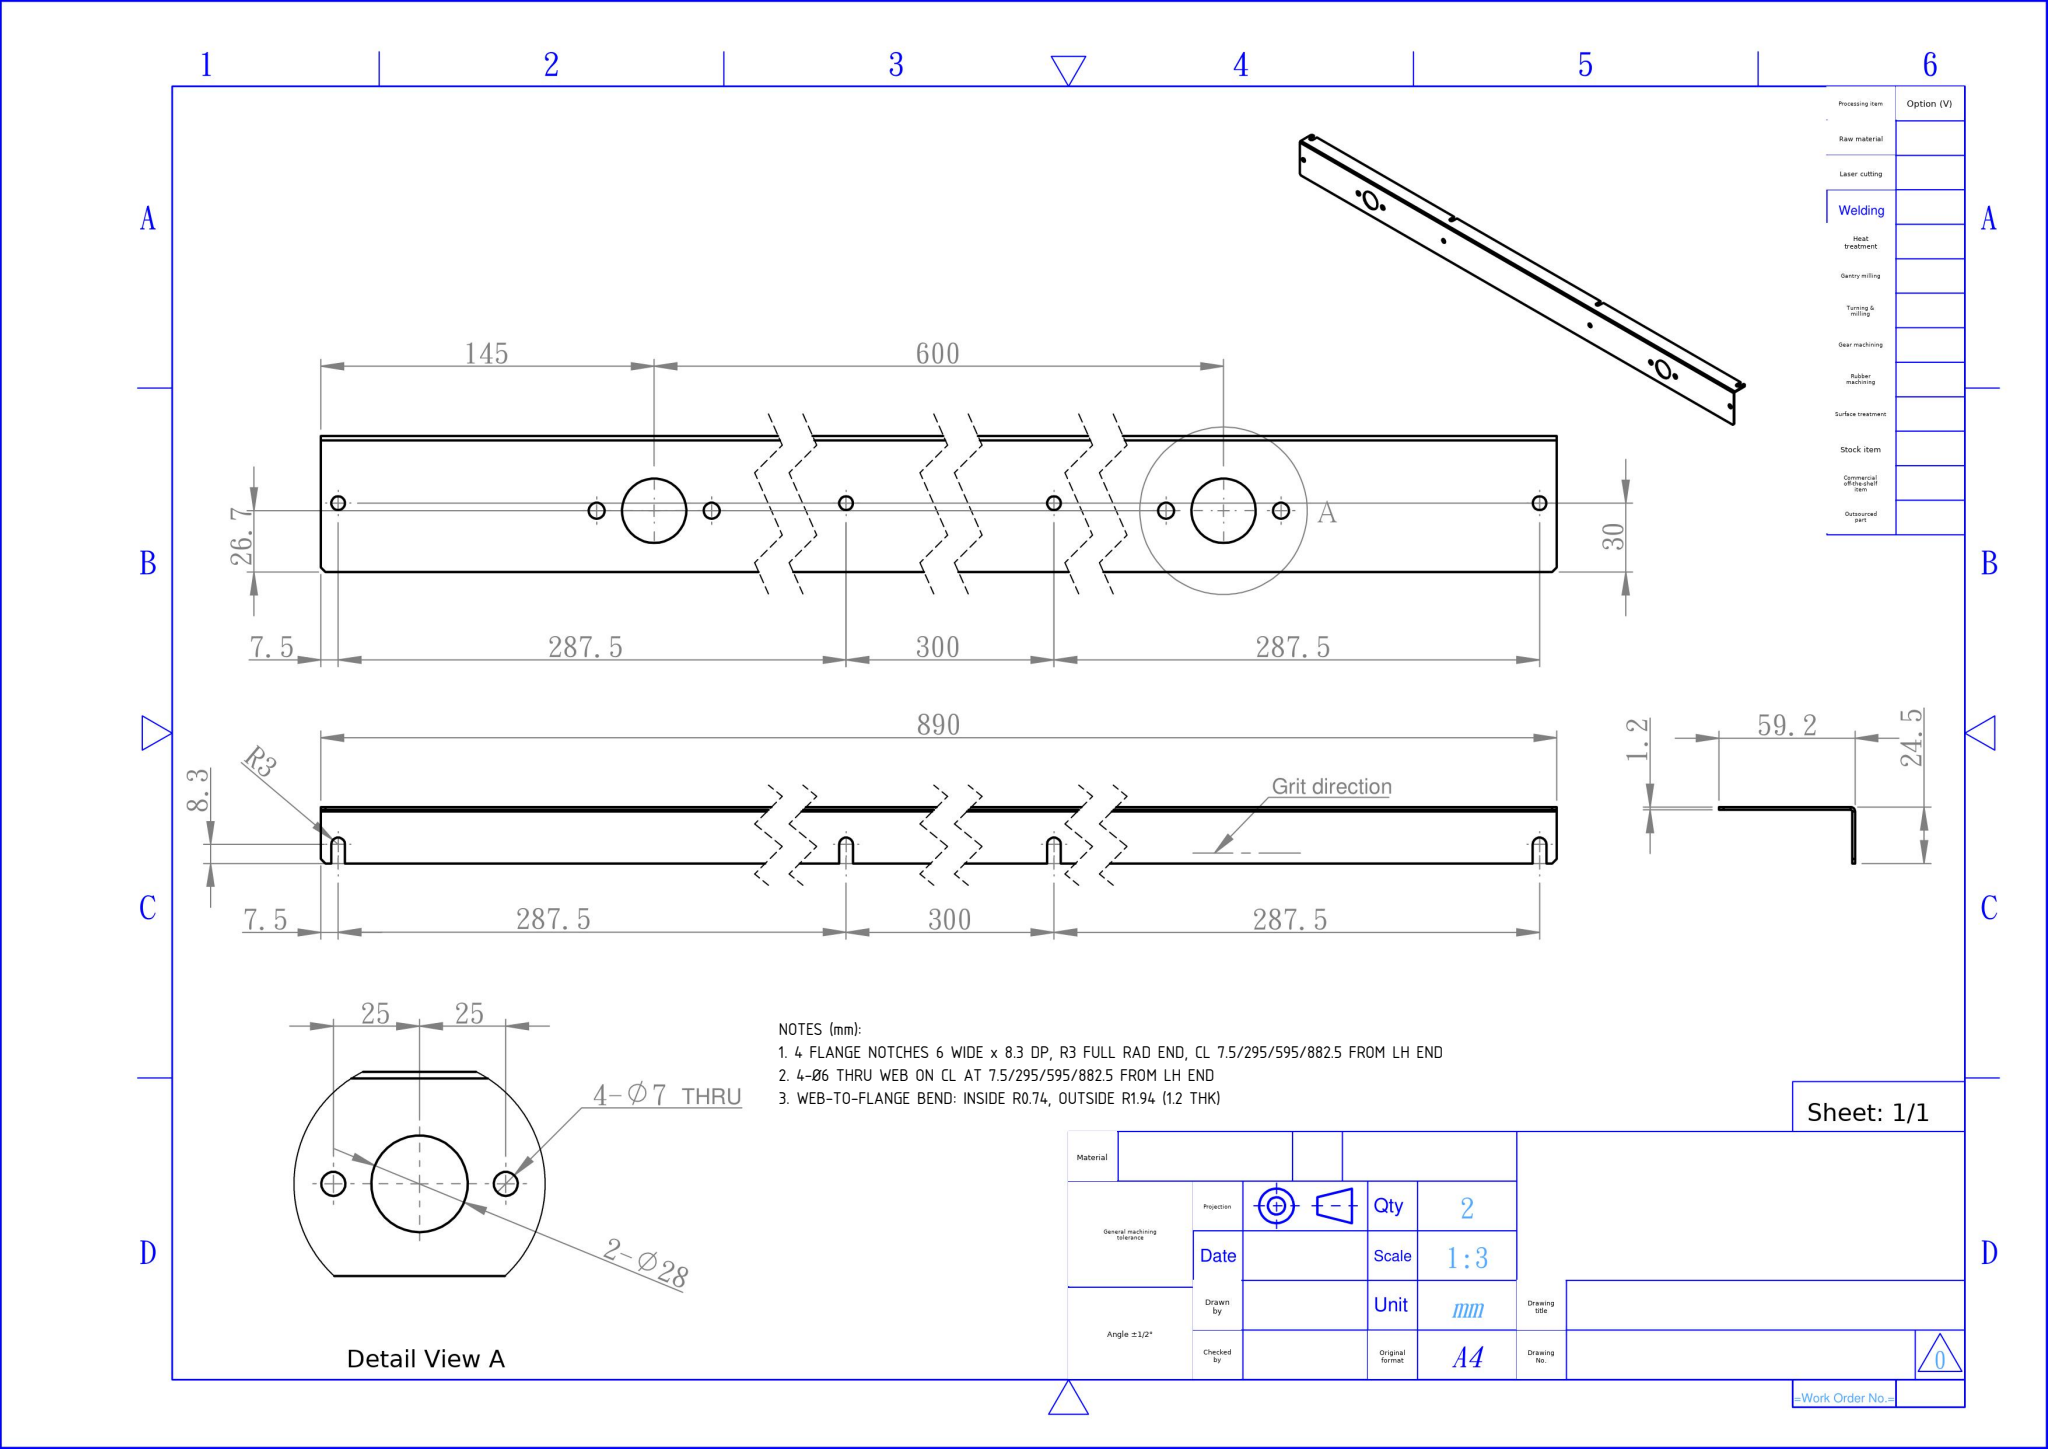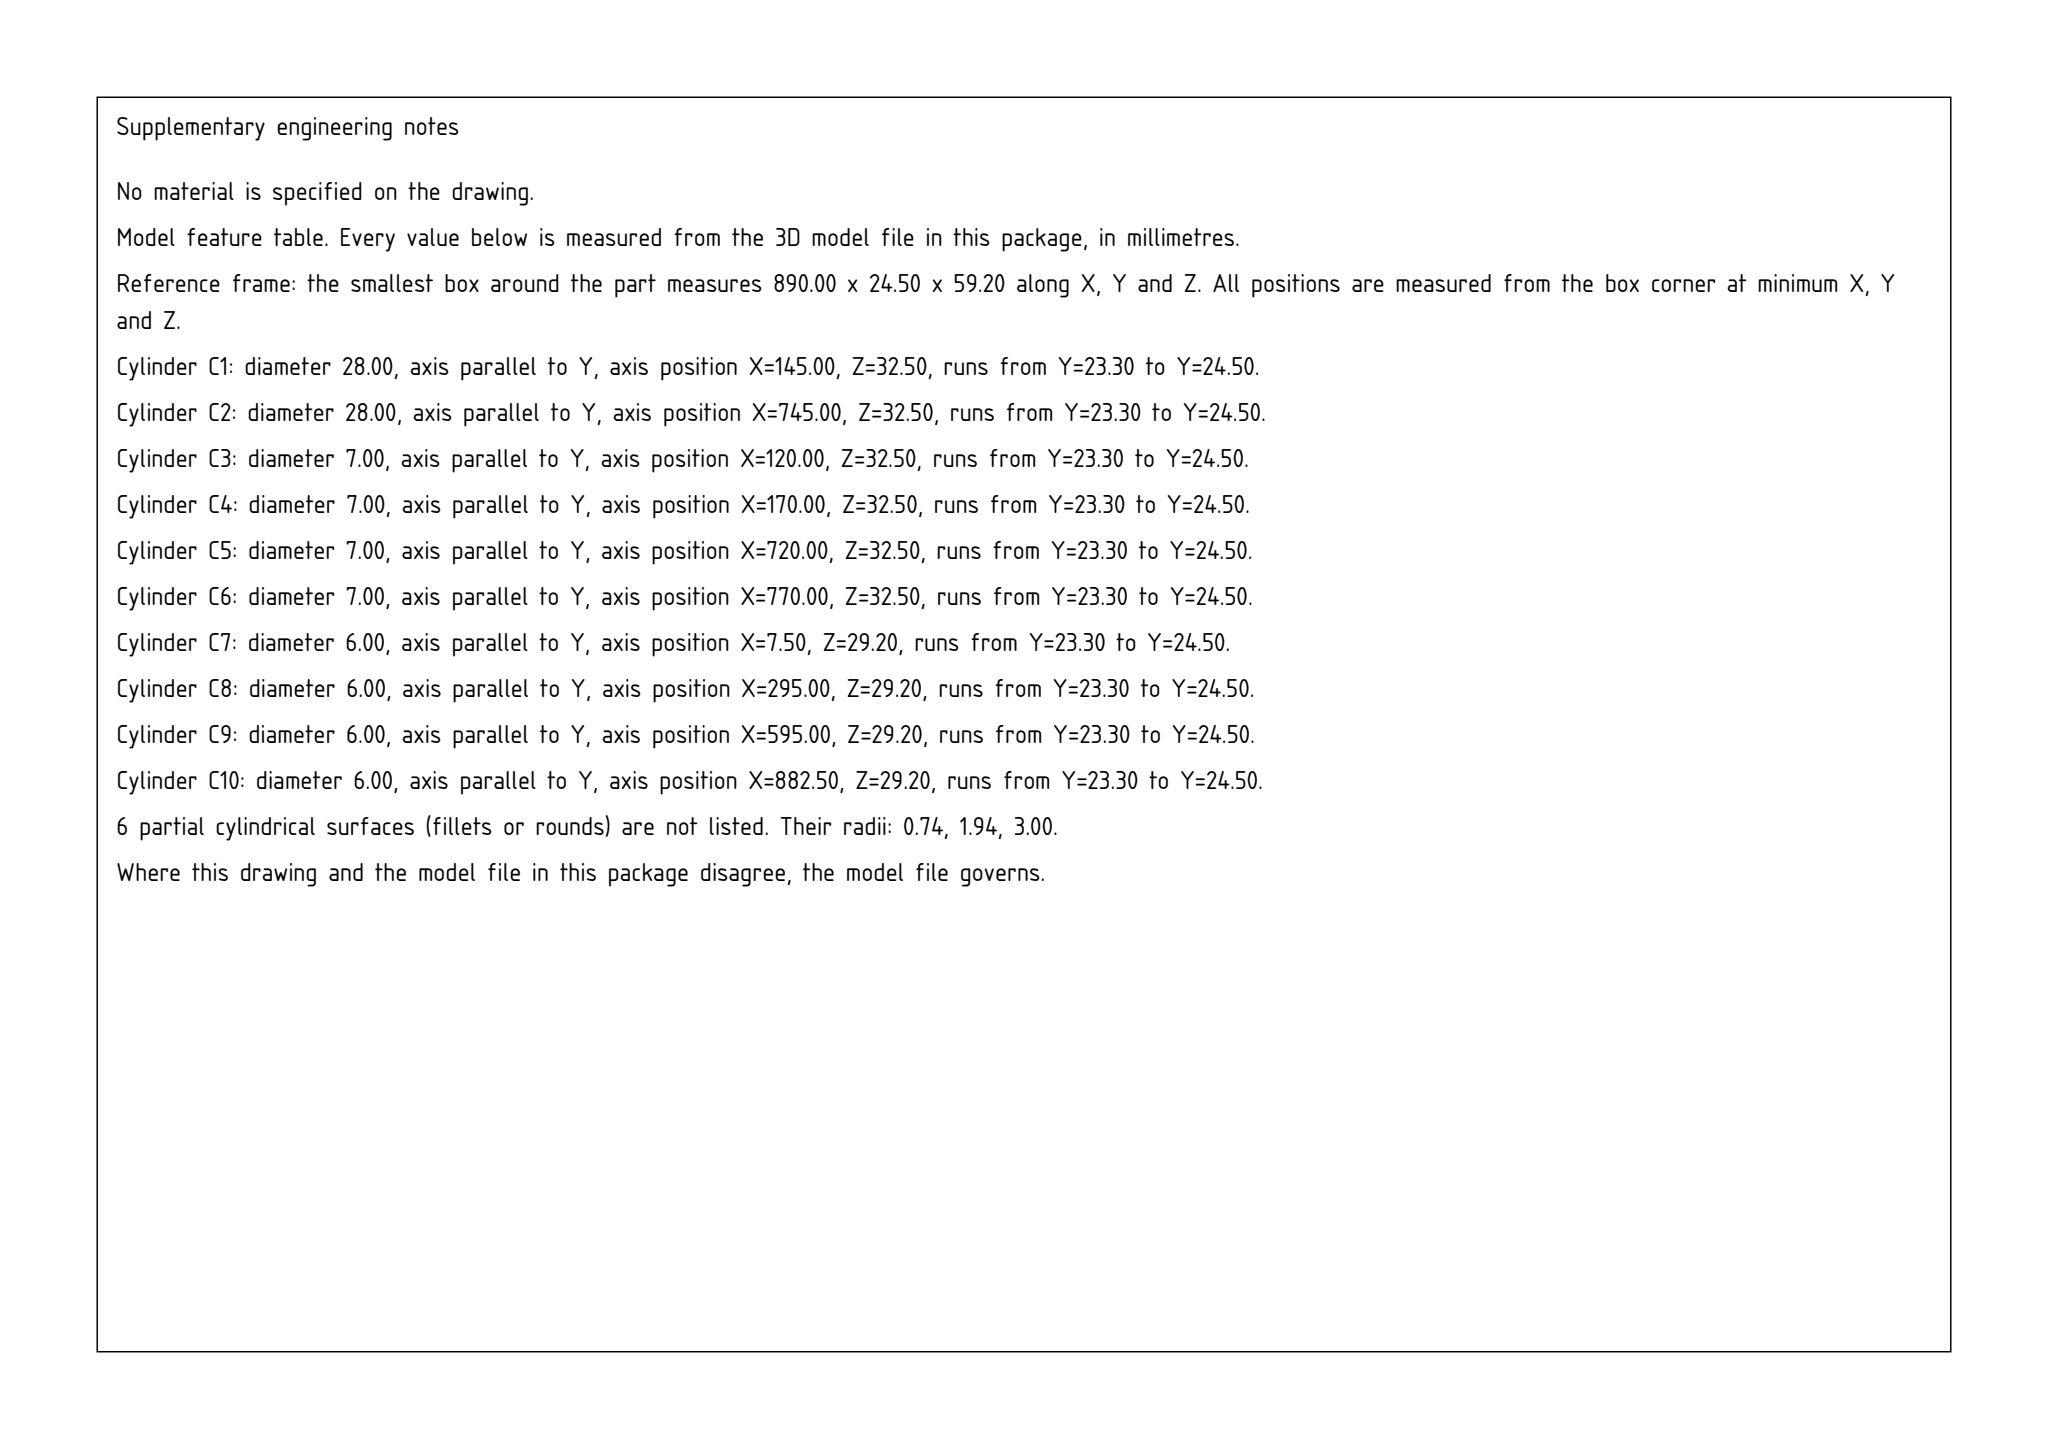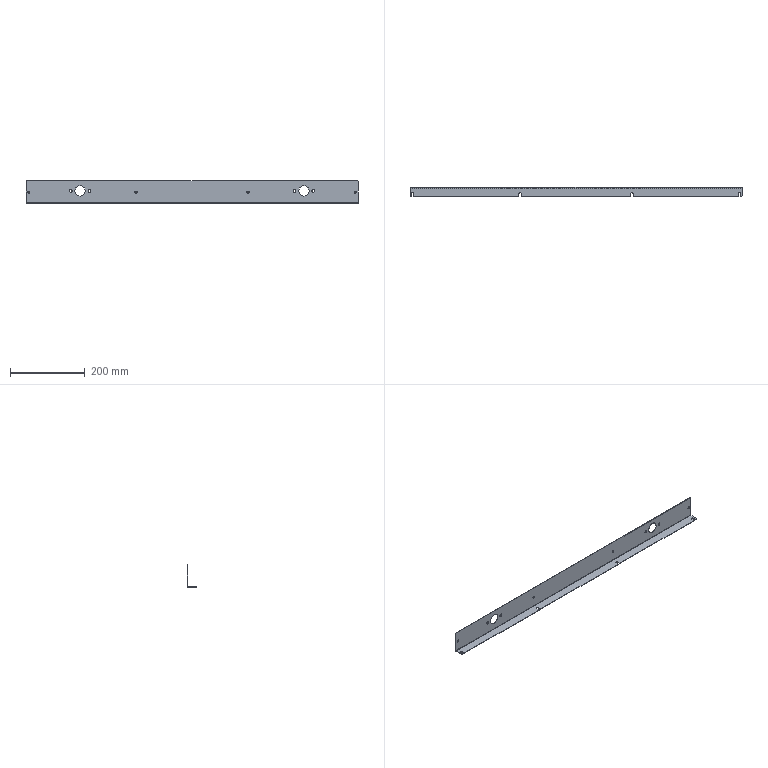Part | SolidWorks | mm | 1 solid | 58 faces | box 890 x 24.5 x 59.2 mm | volume 85383 mm3 | cylinder 30 | plane 28 | commonest cylinder face diameters 6 x16 7 x8 28 x4 3.873 x1 1.473 x1
Drawing notes:
4 FLANGE NOTCHES 6 WIDE x 8.3 DP, R3 FULL RAD END, CL 7.5/295/595/882.5 FROM LH END | from the solid: x-planes 4.5/10.5, 292/298, 592/598, 879.5/885.5 = 6 wide; Ø6 z-axis cyl at y=8.3 = R3 end
4-Ø6 THRU WEB ON CL AT 7.5/295/595/882.5 FROM LH END | from the solid: cylinders dia 6.0 axis y at x=7.5,295,595,882.5, z=29.2, length 1.2 (web thk)
WEB-TO-FLANGE BEND: INSIDE R0.74, OUTSIDE R1.94 (1.2 THK) | from the solid: cyl dia 1.473 & 3.873 abt X axis at (y=22.56,z=1.94), L=890; 1.937-0.7365=1.2 thk